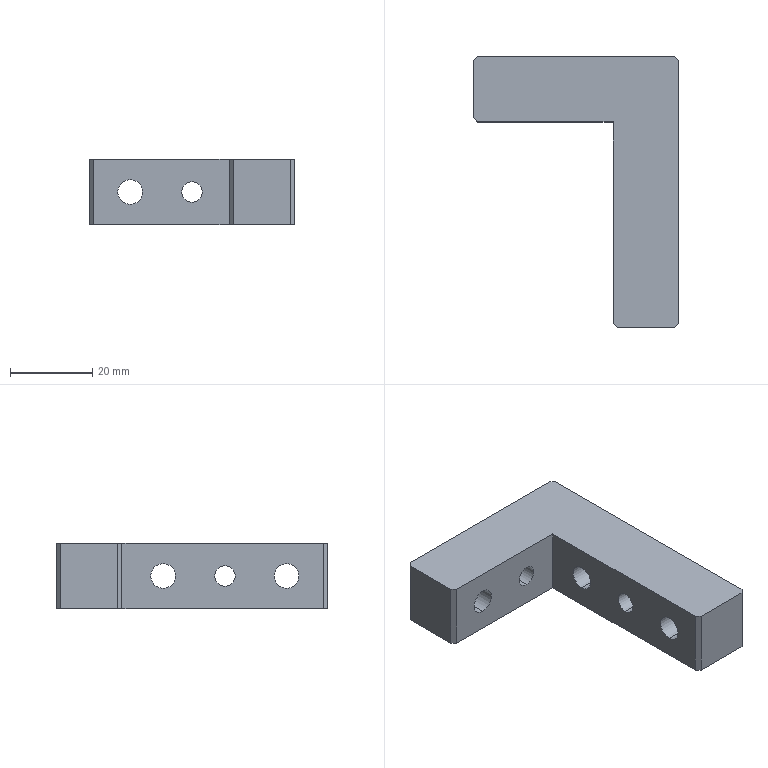Component | SolidWorks | AdjustmentSeat001-1 | 1 solid | 27 faces | box 50 x 66 x 16 mm | volume 22992 mm3 | plane 13 | cylinder 12 | cone 2 | commonest cylinder face diameters 6 x8 5 x4 | material Plain Carbon Steel
build123d program:
from build123d import *

# Parameters (mm, degrees)
EXTRUDE_THIN1_DEPTH          = 8
M6_TAPPED_HOLE2_D            = 5
M6_TAPPED_HOLE2_DEPTH        = 21
M6_TAPPED_HOLE2_TIP          = 1.502
F_6_0_6_DIAMETER_HOLE1_D     = 6
M6_TAPPED_HOLE1_D            = 5
F_6_0_6_DIAMETER_HOLE2_D     = 6
F_6_0_6_DIAMETER_HOLE2_DEPTH = 20
F_6_0_6_DIAMETER_HOLE2_TIP   = 1.803
CHAMFER1_SIZE                = 1


with BuildPart() as part:
    # Sketch1 → Extrude-Thin1 (new, symmetric)
    with BuildSketch(Plane.XY):
        Polygon((0, 34), (0, 0), (-50, 0), (-50, -16), (16, -16), (16, 34), align=None)
    extrude(amount=EXTRUDE_THIN1_DEPTH, both=True)

    # M6 Tapped Hole2
    with Locations(Plane(origin=(0, 0, 0), x_dir=(1, 0, 0), z_dir=(0, 1, 0))):
        with Locations((-25, 0)):
            Hole(M6_TAPPED_HOLE2_D / 2, depth=M6_TAPPED_HOLE2_DEPTH)
            with Locations((0, 0, -(M6_TAPPED_HOLE2_DEPTH + M6_TAPPED_HOLE2_TIP / 2))):  # 118° drill point
                Cone(0, M6_TAPPED_HOLE2_D / 2, M6_TAPPED_HOLE2_TIP, mode=Mode.SUBTRACT)

    # 6.0 _6_ Diameter Hole1 (through all)
    with Locations(Plane(origin=(0, 0, 0), x_dir=(1, 0, 0), z_dir=(0, 1, 0))):
        with Locations((-40, 0), (-10, 0)):
            Hole(F_6_0_6_DIAMETER_HOLE1_D / 2)

    # M6 Tapped Hole1 (through all)
    with Locations(Plane(origin=(16, 0, 0), x_dir=(0, 0, -1), z_dir=(1, 0, 0))):
        with Locations((0, 9)):
            Hole(M6_TAPPED_HOLE1_D / 2)

    # 6.0 _6_ Diameter Hole2
    with Locations(Plane(origin=(16, 0, 0), x_dir=(0, 0, -1), z_dir=(1, 0, 0))):
        with Locations((0, -6), (0, 24)):
            Hole(F_6_0_6_DIAMETER_HOLE2_D / 2, depth=F_6_0_6_DIAMETER_HOLE2_DEPTH)
            with Locations((0, 0, -(F_6_0_6_DIAMETER_HOLE2_DEPTH + F_6_0_6_DIAMETER_HOLE2_TIP / 2))):  # 118° drill point
                Cone(0, F_6_0_6_DIAMETER_HOLE2_D / 2, F_6_0_6_DIAMETER_HOLE2_TIP, mode=Mode.SUBTRACT)

    # Chamfer1
    chamfer1_edges = [part.edges().sort_by_distance(p)[0] for p in [
        (16, -16, 0),
        (-50, -16, 0),
        (-50, 0, 0),
        (0, 34, 0),
        (16, 34, 0),
    ]]
    chamfer(chamfer1_edges, length=CHAMFER1_SIZE)


solid = part.part

# Placed as in the assembly
solid = solid.moved(Location((-17.972, 9.101, 117.932), (0, 0, 90)))
STEP:
#1=COLOUR_RGB('',0.7922,0.8196,0.9333);
#2=FILL_AREA_STYLE_COLOUR('',#1);
#3=FILL_AREA_STYLE('',(#2));
#4=SURFACE_STYLE_FILL_AREA(#3);
#5=SURFACE_SIDE_STYLE('',(#4));
#6=SURFACE_STYLE_USAGE(.BOTH.,#5);
#7=PRESENTATION_STYLE_ASSIGNMENT((#6));
#8=CARTESIAN_POINT('',(-0.4713,0.2008,4.761));
#9=VERTEX_POINT('',#8);
#10=CARTESIAN_POINT('',(-0.4713,0.2008,4.525));
#11=VERTEX_POINT('',#10);
#12=CARTESIAN_POINT('',(-0.4713,0.2008,4.643));
#13=DIRECTION('',(-0.,1.,0.));
#14=DIRECTION('',(0.,0.,-1.));
#15=AXIS2_PLACEMENT_3D('',#12,#13,#14);
#16=CIRCLE('',#15,0.1181);
#17=EDGE_CURVE('',#9,#11,#16,.T.);
#18=ORIENTED_EDGE('',*,*,#17,.F.);
#19=CARTESIAN_POINT('',(-0.4713,0.9882,4.761));
#20=VERTEX_POINT('',#19);
#21=CARTESIAN_POINT('',(-0.4713,0.9882,4.761));
#22=DIRECTION('',(-0.,1.,0.));
#23=VECTOR('',#22,39.37);
#24=LINE('',#21,#23);
#25=EDGE_CURVE('',#9,#20,#24,.T.);
#26=ORIENTED_EDGE('',*,*,#25,.T.);
#27=CARTESIAN_POINT('',(-0.4713,0.9882,4.525));
#28=VERTEX_POINT('',#27);
#29=CARTESIAN_POINT('',(-0.4713,0.9882,4.643));
#30=DIRECTION('',(-0.,1.,0.));
#31=DIRECTION('',(0.,0.,-1.));
#32=AXIS2_PLACEMENT_3D('',#29,#30,#31);
#33=CIRCLE('',#32,0.1181);
#34=EDGE_CURVE('',#20,#28,#33,.T.);
#35=ORIENTED_EDGE('',*,*,#34,.T.);
#36=CARTESIAN_POINT('',(-0.4713,0.9882,4.525));
#37=DIRECTION('',(-0.,1.,0.));
#38=VECTOR('',#37,39.37);
#39=LINE('',#36,#38);
#40=EDGE_CURVE('',#11,#28,#39,.T.);
#41=ORIENTED_EDGE('',*,*,#40,.F.);
#42=EDGE_LOOP('',(#18,#26,#35,#41));
#43=FACE_OUTER_BOUND('',#42,.T.);
#44=CARTESIAN_POINT('',(-0.4713,0.9882,4.643));
#45=DIRECTION('',(-0.,1.,0.));
#46=DIRECTION('',(0.,0.,-1.));
#47=AXIS2_PLACEMENT_3D('',#44,#45,#46);
#48=CYLINDRICAL_SURFACE('',#47,0.1181);
#49=ADVANCED_FACE('',(#43),#48,.F.);
#50=CARTESIAN_POINT('',(-0.4713,0.1299,4.643));
#51=VERTEX_POINT('',#50);
#52=CARTESIAN_POINT('',(-0.4713,0.2008,4.525));
#53=DIRECTION('',(-0.,0.515,-0.8572));
#54=VECTOR('',#53,39.37);
#55=LINE('',#52,#54);
#56=EDGE_CURVE('',#51,#11,#55,.T.);
#57=ORIENTED_EDGE('',*,*,#56,.F.);
#58=CARTESIAN_POINT('',(-0.4713,0.2008,4.761));
#59=DIRECTION('',(-0.,0.515,0.8572));
#60=VECTOR('',#59,39.37);
#61=LINE('',#58,#60);
#62=EDGE_CURVE('',#51,#9,#61,.T.);
#63=ORIENTED_EDGE('',*,*,#62,.T.);
#64=ORIENTED_EDGE('',*,*,#17,.T.);
#65=EDGE_LOOP('',(#57,#63,#64));
#66=FACE_OUTER_BOUND('',#65,.T.);
#67=CARTESIAN_POINT('',(-0.4713,0.2008,4.643));
#68=DIRECTION('',(-0.,1.,0.));
#69=DIRECTION('',(0.,0.,-1.));
#70=AXIS2_PLACEMENT_3D('',#67,#68,#69);
#71=CONICAL_SURFACE('',#70,0.1181,1.03);
#72=ADVANCED_FACE('',(#66),#71,.F.);
#73=CARTESIAN_POINT('',(-1.652,0.3583,4.525));
#74=VERTEX_POINT('',#73);
#75=CARTESIAN_POINT('',(-1.652,0.3583,4.761));
#76=VERTEX_POINT('',#75);
#77=CARTESIAN_POINT('',(-1.652,0.3583,4.643));
#78=DIRECTION('',(0.,-1.,0.));
#79=DIRECTION('',(0.,0.,1.));
#80=AXIS2_PLACEMENT_3D('',#77,#78,#79);
#81=CIRCLE('',#80,0.1181);
#82=EDGE_CURVE('',#74,#76,#81,.T.);
#83=ORIENTED_EDGE('',*,*,#82,.T.);
#84=CARTESIAN_POINT('',(-1.652,0.9882,4.761));
#85=VERTEX_POINT('',#84);
#86=CARTESIAN_POINT('',(-1.652,0.9882,4.761));
#87=DIRECTION('',(-0.,1.,0.));
#88=VECTOR('',#87,39.37);
#89=LINE('',#86,#88);
#90=EDGE_CURVE('',#76,#85,#89,.T.);
#91=ORIENTED_EDGE('',*,*,#90,.T.);
#92=CARTESIAN_POINT('',(-1.652,0.9882,4.525));
#93=VERTEX_POINT('',#92);
#94=CARTESIAN_POINT('',(-1.652,0.9882,4.643));
#95=DIRECTION('',(-0.,1.,0.));
#96=DIRECTION('',(0.,0.,-1.));
#97=AXIS2_PLACEMENT_3D('',#94,#95,#96);
#98=CIRCLE('',#97,0.1181);
#99=EDGE_CURVE('',#85,#93,#98,.T.);
#100=ORIENTED_EDGE('',*,*,#99,.T.);
#101=CARTESIAN_POINT('',(-1.652,0.9882,4.525));
#102=DIRECTION('',(-0.,1.,0.));
#103=VECTOR('',#102,39.37);
#104=LINE('',#101,#103);
#105=EDGE_CURVE('',#74,#93,#104,.T.);
#106=ORIENTED_EDGE('',*,*,#105,.F.);
#107=EDGE_LOOP('',(#83,#91,#100,#106));
#108=FACE_OUTER_BOUND('',#107,.T.);
#109=CARTESIAN_POINT('',(-1.652,0.9882,4.643));
#110=DIRECTION('',(-0.,1.,0.));
#111=DIRECTION('',(0.,0.,-1.));
#112=AXIS2_PLACEMENT_3D('',#109,#110,#111);
#113=CYLINDRICAL_SURFACE('',#112,0.1181);
#114=ADVANCED_FACE('',(#108),#113,.F.);
#115=CARTESIAN_POINT('',(-1.062,0.3583,4.545));
#116=VERTEX_POINT('',#115);
#117=CARTESIAN_POINT('',(-1.062,0.3583,4.741));
#118=VERTEX_POINT('',#117);
#119=CARTESIAN_POINT('',(-1.062,0.3583,4.643));
#120=DIRECTION('',(0.,-1.,0.));
#121=DIRECTION('',(0.,0.,1.));
#122=AXIS2_PLACEMENT_3D('',#119,#120,#121);
#123=CIRCLE('',#122,0.09843);
#124=EDGE_CURVE('',#116,#118,#123,.T.);
#125=ORIENTED_EDGE('',*,*,#124,.T.);
#126=CARTESIAN_POINT('',(-1.062,0.9882,4.741));
#127=VERTEX_POINT('',#126);
#128=CARTESIAN_POINT('',(-1.062,0.9882,4.741));
#129=DIRECTION('',(-0.,1.,0.));
#130=VECTOR('',#129,39.37);
#131=LINE('',#128,#130);
#132=EDGE_CURVE('',#118,#127,#131,.T.);
#133=ORIENTED_EDGE('',*,*,#132,.T.);
#134=CARTESIAN_POINT('',(-1.062,0.9882,4.545));
#135=VERTEX_POINT('',#134);
#136=CARTESIAN_POINT('',(-1.062,0.9882,4.643));
#137=DIRECTION('',(-0.,1.,0.));
#138=DIRECTION('',(0.,0.,-1.));
#139=AXIS2_PLACEMENT_3D('',#136,#137,#138);
#140=CIRCLE('',#139,0.09843);
#141=EDGE_CURVE('',#127,#135,#140,.T.);
#142=ORIENTED_EDGE('',*,*,#141,.T.);
#143=CARTESIAN_POINT('',(-1.062,0.9882,4.545));
#144=DIRECTION('',(-0.,1.,0.));
#145=VECTOR('',#144,39.37);
#146=LINE('',#143,#145);
#147=EDGE_CURVE('',#116,#135,#146,.T.);
#148=ORIENTED_EDGE('',*,*,#147,.F.);
#149=EDGE_LOOP('',(#125,#133,#142,#148));
#150=FACE_OUTER_BOUND('',#149,.T.);
#151=CARTESIAN_POINT('',(-1.062,0.9882,4.643));
#152=DIRECTION('',(-0.,1.,0.));
#153=DIRECTION('',(0.,0.,-1.));
#154=AXIS2_PLACEMENT_3D('',#151,#152,#153);
#155=CYLINDRICAL_SURFACE('',#154,0.09843);
#156=ADVANCED_FACE('',(#150),#155,.F.);
#157=CARTESIAN_POINT('',(-0.07764,-1.216,4.525));
#158=VERTEX_POINT('',#157);
#159=CARTESIAN_POINT('',(-0.07764,-1.216,4.761));
#160=VERTEX_POINT('',#159);
#161=CARTESIAN_POINT('',(-0.07764,-1.216,4.643));
#162=DIRECTION('',(-1.,-0.,0.));
#163=DIRECTION('',(0.,0.,1.));
#164=AXIS2_PLACEMENT_3D('',#161,#162,#163);
#165=CIRCLE('',#164,0.1181);
#166=EDGE_CURVE('',#158,#160,#165,.T.);
#167=ORIENTED_EDGE('',*,*,#166,.F.);
#168=CARTESIAN_POINT('',(-0.7076,-1.216,4.525));
#169=VERTEX_POINT('',#168);
#170=CARTESIAN_POINT('',(-0.7076,-1.216,4.525));
#171=DIRECTION('',(-1.,-0.,0.));
#172=VECTOR('',#171,39.37);
#173=LINE('',#170,#172);
#174=EDGE_CURVE('',#158,#169,#173,.T.);
#175=ORIENTED_EDGE('',*,*,#174,.T.);
#176=CARTESIAN_POINT('',(-0.7076,-1.216,4.761));
#177=VERTEX_POINT('',#176);
#178=CARTESIAN_POINT('',(-0.7076,-1.216,4.643));
#179=DIRECTION('',(-1.,-0.,0.));
#180=DIRECTION('',(0.,0.,1.));
#181=AXIS2_PLACEMENT_3D('',#178,#179,#180);
#182=CIRCLE('',#181,0.1181);
#183=EDGE_CURVE('',#169,#177,#182,.T.);
#184=ORIENTED_EDGE('',*,*,#183,.T.);
#185=CARTESIAN_POINT('',(-0.7076,-1.216,4.761));
#186=DIRECTION('',(-1.,-0.,0.));
#187=VECTOR('',#186,39.37);
#188=LINE('',#185,#187);
#189=EDGE_CURVE('',#160,#177,#188,.T.);
#190=ORIENTED_EDGE('',*,*,#189,.F.);
#191=EDGE_LOOP('',(#167,#175,#184,#190));
#192=FACE_OUTER_BOUND('',#191,.T.);
#193=CARTESIAN_POINT('',(-0.7076,-1.216,4.643));
#194=DIRECTION('',(-1.,-0.,0.));
#195=DIRECTION('',(0.,0.,1.));
#196=AXIS2_PLACEMENT_3D('',#193,#194,#195);
#197=CYLINDRICAL_SURFACE('',#196,0.1181);
#198=ADVANCED_FACE('',(#192),#197,.F.);
#199=CARTESIAN_POINT('',(-0.07764,-0.03539,4.525));
#200=VERTEX_POINT('',#199);
#201=CARTESIAN_POINT('',(-0.07764,-0.03539,4.761));
#202=VERTEX_POINT('',#201);
#203=CARTESIAN_POINT('',(-0.07764,-0.03539,4.643));
#204=DIRECTION('',(-1.,-0.,0.));
#205=DIRECTION('',(0.,0.,1.));
#206=AXIS2_PLACEMENT_3D('',#203,#204,#205);
#207=CIRCLE('',#206,0.1181);
#208=EDGE_CURVE('',#200,#202,#207,.T.);
#209=ORIENTED_EDGE('',*,*,#208,.F.);
#210=CARTESIAN_POINT('',(-0.7076,-0.03539,4.525));
#211=VERTEX_POINT('',#210);
#212=CARTESIAN_POINT('',(-0.7076,-0.03539,4.525));
#213=DIRECTION('',(-1.,-0.,0.));
#214=VECTOR('',#213,39.37);
#215=LINE('',#212,#214);
#216=EDGE_CURVE('',#200,#211,#215,.T.);
#217=ORIENTED_EDGE('',*,*,#216,.T.);
#218=CARTESIAN_POINT('',(-0.7076,-0.03539,4.761));
#219=VERTEX_POINT('',#218);
#220=CARTESIAN_POINT('',(-0.7076,-0.03539,4.643));
#221=DIRECTION('',(-1.,-0.,0.));
#222=DIRECTION('',(0.,0.,1.));
#223=AXIS2_PLACEMENT_3D('',#220,#221,#222);
#224=CIRCLE('',#223,0.1181);
#225=EDGE_CURVE('',#211,#219,#224,.T.);
#226=ORIENTED_EDGE('',*,*,#225,.T.);
#227=CARTESIAN_POINT('',(-0.7076,-0.03539,4.761));
#228=DIRECTION('',(-1.,-0.,0.));
#229=VECTOR('',#228,39.37);
#230=LINE('',#227,#229);
#231=EDGE_CURVE('',#202,#219,#230,.T.);
#232=ORIENTED_EDGE('',*,*,#231,.F.);
#233=EDGE_LOOP('',(#209,#217,#226,#232));
#234=FACE_OUTER_BOUND('',#233,.T.);
#235=CARTESIAN_POINT('',(-0.7076,-0.03539,4.643));
#236=DIRECTION('',(-1.,-0.,0.));
#237=DIRECTION('',(0.,0.,1.));
#238=AXIS2_PLACEMENT_3D('',#235,#236,#237);
#239=CYLINDRICAL_SURFACE('',#238,0.1181);
#240=ADVANCED_FACE('',(#234),#239,.F.);
#241=CARTESIAN_POINT('',(-0.07764,-0.6259,4.545));
#242=VERTEX_POINT('',#241);
#243=CARTESIAN_POINT('',(-0.07764,-0.6259,4.741));
#244=VERTEX_POINT('',#243);
#245=CARTESIAN_POINT('',(-0.07764,-0.6259,4.643));
#246=DIRECTION('',(-1.,-0.,0.));
#247=DIRECTION('',(0.,0.,1.));
#248=AXIS2_PLACEMENT_3D('',#245,#246,#247);
#249=CIRCLE('',#248,0.09843);
#250=EDGE_CURVE('',#242,#244,#249,.T.);
#251=ORIENTED_EDGE('',*,*,#250,.F.);
#252=CARTESIAN_POINT('',(-0.7076,-0.6259,4.545));
#253=VERTEX_POINT('',#252);
#254=CARTESIAN_POINT('',(-0.7076,-0.6259,4.545));
#255=DIRECTION('',(-1.,-0.,0.));
#256=VECTOR('',#255,39.37);
#257=LINE('',#254,#256);
#258=EDGE_CURVE('',#242,#253,#257,.T.);
#259=ORIENTED_EDGE('',*,*,#258,.T.);
#260=CARTESIAN_POINT('',(-0.7076,-0.6259,4.741));
#261=VERTEX_POINT('',#260);
#262=CARTESIAN_POINT('',(-0.7076,-0.6259,4.643));
#263=DIRECTION('',(-1.,-0.,0.));
#264=DIRECTION('',(0.,0.,1.));
#265=AXIS2_PLACEMENT_3D('',#262,#263,#264);
#266=CIRCLE('',#265,0.09843);
#267=EDGE_CURVE('',#253,#261,#266,.T.);
#268=ORIENTED_EDGE('',*,*,#267,.T.);
#269=CARTESIAN_POINT('',(-0.7076,-0.6259,4.741));
#270=DIRECTION('',(-1.,-0.,0.));
#271=VECTOR('',#270,39.37);
#272=LINE('',#269,#271);
#273=EDGE_CURVE('',#244,#261,#272,.T.);
#274=ORIENTED_EDGE('',*,*,#273,.F.);
#275=EDGE_LOOP('',(#251,#259,#268,#274));
#276=FACE_OUTER_BOUND('',#275,.T.);
#277=CARTESIAN_POINT('',(-0.7076,-0.6259,4.643));
#278=DIRECTION('',(-1.,-0.,0.));
#279=DIRECTION('',(0.,0.,1.));
#280=AXIS2_PLACEMENT_3D('',#277,#278,#279);
#281=CYLINDRICAL_SURFACE('',#280,0.09843);
#282=ADVANCED_FACE('',(#276),#281,.F.);
#283=CARTESIAN_POINT('',(-0.4713,0.9882,4.643));
#284=DIRECTION('',(-0.,1.,0.));
#285=DIRECTION('',(0.,0.,-1.));
#286=AXIS2_PLACEMENT_3D('',#283,#284,#285);
#287=CIRCLE('',#286,0.1181);
#288=EDGE_CURVE('',#28,#20,#287,.T.);
#289=ORIENTED_EDGE('',*,*,#288,.F.);
#290=ORIENTED_EDGE('',*,*,#34,.F.);
#291=EDGE_LOOP('',(#289,#290));
#292=FACE_BOUND('',#291,.T.);
#293=CARTESIAN_POINT('',(-1.652,0.9882,4.643));
#294=DIRECTION('',(-0.,1.,0.));
#295=DIRECTION('',(0.,0.,-1.));
#296=AXIS2_PLACEMENT_3D('',#293,#294,#295);
#297=CIRCLE('',#296,0.1181);
#298=EDGE_CURVE('',#93,#85,#297,.T.);
#299=ORIENTED_EDGE('',*,*,#298,.F.);
#300=ORIENTED_EDGE('',*,*,#99,.F.);
#301=EDGE_LOOP('',(#299,#300));
#302=FACE_BOUND('',#301,.T.);
#303=CARTESIAN_POINT('',(-1.062,0.9882,4.643));
#304=DIRECTION('',(-0.,1.,0.));
#305=DIRECTION('',(0.,0.,-1.));
#306=AXIS2_PLACEMENT_3D('',#303,#304,#305);
#307=CIRCLE('',#306,0.09843);
#308=EDGE_CURVE('',#135,#127,#307,.T.);
#309=ORIENTED_EDGE('',*,*,#308,.F.);
#310=ORIENTED_EDGE('',*,*,#141,.F.);
#311=EDGE_LOOP('',(#309,#310));
#312=FACE_BOUND('',#311,.T.);
#313=CARTESIAN_POINT('',(-0.117,0.9882,4.958));
#314=VERTEX_POINT('',#313);
#315=CARTESIAN_POINT('',(-2.007,0.9882,4.958));
#316=VERTEX_POINT('',#315);
#317=CARTESIAN_POINT('',(-0.7076,0.9882,4.958));
#318=DIRECTION('',(-1.,-0.,0.));
#319=VECTOR('',#318,39.37);
#320=LINE('',#317,#319);
#321=EDGE_CURVE('',#314,#316,#320,.T.);
#322=ORIENTED_EDGE('',*,*,#321,.F.);
#323=CARTESIAN_POINT('',(-0.117,0.9882,4.328));
#324=VERTEX_POINT('',#323);
#325=CARTESIAN_POINT('',(-0.117,0.9882,4.958));
#326=DIRECTION('',(0.,0.,-1.));
#327=VECTOR('',#326,39.37);
#328=LINE('',#325,#327);
#329=EDGE_CURVE('',#314,#324,#328,.T.);
#330=ORIENTED_EDGE('',*,*,#329,.T.);
#331=CARTESIAN_POINT('',(-2.007,0.9882,4.328));
#332=VERTEX_POINT('',#331);
#333=CARTESIAN_POINT('',(-0.7076,0.9882,4.328));
#334=DIRECTION('',(-1.,-0.,0.));
#335=VECTOR('',#334,39.37);
#336=LINE('',#333,#335);
#337=EDGE_CURVE('',#324,#332,#336,.T.);
#338=ORIENTED_EDGE('',*,*,#337,.T.);
#339=CARTESIAN_POINT('',(-2.007,0.9882,4.958));
#340=DIRECTION('',(0.,0.,1.));
#341=VECTOR('',#340,39.37);
#342=LINE('',#339,#341);
#343=EDGE_CURVE('',#332,#316,#342,.T.);
#344=ORIENTED_EDGE('',*,*,#343,.T.);
#345=EDGE_LOOP('',(#322,#330,#338,#344));
#346=FACE_OUTER_BOUND('',#345,.T.);
#347=CARTESIAN_POINT('',(-0.7076,0.9882,4.958));
#348=DIRECTION('',(0.,-1.,0.));
#349=DIRECTION('',(0.,0.,1.));
#350=AXIS2_PLACEMENT_3D('',#347,#348,#349);
#351=PLANE('',#350);
#352=ADVANCED_FACE('',(#292,#302,#312,#346),#351,.F.);
#353=CARTESIAN_POINT('',(-2.046,0.3977,4.958));
#354=VERTEX_POINT('',#353);
#355=CARTESIAN_POINT('',(-2.046,0.9489,4.958));
#356=VERTEX_POINT('',#355);
#357=CARTESIAN_POINT('',(-2.046,0.3583,4.958));
#358=DIRECTION('',(-0.,1.,0.));
#359=VECTOR('',#358,39.37);
#360=LINE('',#357,#359);
#361=EDGE_CURVE('',#354,#356,#360,.T.);
#362=ORIENTED_EDGE('',*,*,#361,.T.);
#363=CARTESIAN_POINT('',(-2.046,0.9489,4.328));
#364=VERTEX_POINT('',#363);
#365=CARTESIAN_POINT('',(-2.046,0.9489,4.328));
#366=DIRECTION('',(0.,0.,-1.));
#367=VECTOR('',#366,39.37);
#368=LINE('',#365,#367);
#369=EDGE_CURVE('',#356,#364,#368,.T.);
#370=ORIENTED_EDGE('',*,*,#369,.T.);
#371=CARTESIAN_POINT('',(-2.046,0.3977,4.328));
#372=VERTEX_POINT('',#371);
#373=CARTESIAN_POINT('',(-2.046,0.3583,4.328));
#374=DIRECTION('',(-0.,1.,0.));
#375=VECTOR('',#374,39.37);
#376=LINE('',#373,#375);
#377=EDGE_CURVE('',#372,#364,#376,.T.);
#378=ORIENTED_EDGE('',*,*,#377,.F.);
#379=CARTESIAN_POINT('',(-2.046,0.3977,4.958));
#380=DIRECTION('',(0.,0.,1.));
#381=VECTOR('',#380,39.37);
#382=LINE('',#379,#381);
#383=EDGE_CURVE('',#372,#354,#382,.T.);
#384=ORIENTED_EDGE('',*,*,#383,.T.);
#385=EDGE_LOOP('',(#362,#370,#378,#384));
#386=FACE_OUTER_BOUND('',#385,.T.);
#387=CARTESIAN_POINT('',(-2.046,0.3583,4.958));
#388=DIRECTION('',(-1.,-0.,0.));
#389=DIRECTION('',(0.,0.,1.));
#390=AXIS2_PLACEMENT_3D('',#387,#388,#389);
#391=PLANE('',#390);
#392=ADVANCED_FACE('',(#386),#391,.T.);
#393=ORIENTED_EDGE('',*,*,#82,.F.);
#394=CARTESIAN_POINT('',(-1.652,0.3583,4.643));
#395=DIRECTION('',(0.,-1.,0.));
#396=DIRECTION('',(0.,0.,1.));
#397=AXIS2_PLACEMENT_3D('',#394,#395,#396);
#398=CIRCLE('',#397,0.1181);
#399=EDGE_CURVE('',#76,#74,#398,.T.);
#400=ORIENTED_EDGE('',*,*,#399,.F.);
#401=EDGE_LOOP('',(#393,#400));
#402=FACE_BOUND('',#401,.T.);
#403=ORIENTED_EDGE('',*,*,#124,.F.);
#404=CARTESIAN_POINT('',(-1.062,0.3583,4.643));
#405=DIRECTION('',(0.,-1.,0.));
#406=DIRECTION('',(0.,0.,1.));
#407=AXIS2_PLACEMENT_3D('',#404,#405,#406);
#408=CIRCLE('',#407,0.09843);
#409=EDGE_CURVE('',#118,#116,#408,.T.);
#410=ORIENTED_EDGE('',*,*,#409,.F.);
#411=EDGE_LOOP('',(#403,#410));
#412=FACE_BOUND('',#411,.T.);
#413=CARTESIAN_POINT('',(-0.7076,0.3583,4.958));
#414=VERTEX_POINT('',#413);
#415=CARTESIAN_POINT('',(-2.007,0.3583,4.958));
#416=VERTEX_POINT('',#415);
#417=CARTESIAN_POINT('',(-0.7076,0.3583,4.958));
#418=DIRECTION('',(-1.,-0.,0.));
#419=VECTOR('',#418,39.37);
#420=LINE('',#417,#419);
#421=EDGE_CURVE('',#414,#416,#420,.T.);
#422=ORIENTED_EDGE('',*,*,#421,.T.);
#423=CARTESIAN_POINT('',(-2.007,0.3583,4.328));
#424=VERTEX_POINT('',#423);
#425=CARTESIAN_POINT('',(-2.007,0.3583,4.958));
#426=DIRECTION('',(0.,0.,-1.));
#427=VECTOR('',#426,39.37);
#428=LINE('',#425,#427);
#429=EDGE_CURVE('',#416,#424,#428,.T.);
#430=ORIENTED_EDGE('',*,*,#429,.T.);
#431=CARTESIAN_POINT('',(-0.7076,0.3583,4.328));
#432=VERTEX_POINT('',#431);
#433=CARTESIAN_POINT('',(-0.7076,0.3583,4.328));
#434=DIRECTION('',(-1.,-0.,0.));
#435=VECTOR('',#434,39.37);
#436=LINE('',#433,#435);
#437=EDGE_CURVE('',#432,#424,#436,.T.);
#438=ORIENTED_EDGE('',*,*,#437,.F.);
#439=CARTESIAN_POINT('',(-0.7076,0.3583,4.958));
#440=DIRECTION('',(0.,0.,-1.));
#441=VECTOR('',#440,39.37);
#442=LINE('',#439,#441);
#443=EDGE_CURVE('',#414,#432,#442,.T.);
#444=ORIENTED_EDGE('',*,*,#443,.F.);
#445=EDGE_LOOP('',(#422,#430,#438,#444));
#446=FACE_OUTER_BOUND('',#445,.T.);
#447=CARTESIAN_POINT('',(-0.7076,0.3583,4.958));
#448=DIRECTION('',(0.,-1.,0.));
#449=DIRECTION('',(0.,0.,1.));
#450=AXIS2_PLACEMENT_3D('',#447,#448,#449);
#451=PLANE('',#450);
#452=ADVANCED_FACE('',(#402,#412,#446),#451,.T.);
#453=CARTESIAN_POINT('',(-0.7076,-1.216,4.643));
#454=DIRECTION('',(-1.,-0.,0.));
#455=DIRECTION('',(0.,0.,1.));
#456=AXIS2_PLACEMENT_3D('',#453,#454,#455);
#457=CIRCLE('',#456,0.1181);
#458=EDGE_CURVE('',#177,#169,#457,.T.);
#459=ORIENTED_EDGE('',*,*,#458,.F.);
#460=ORIENTED_EDGE('',*,*,#183,.F.);
#461=EDGE_LOOP('',(#459,#460));
#462=FACE_BOUND('',#461,.T.);
#463=CARTESIAN_POINT('',(-0.7076,-0.03539,4.643));
#464=DIRECTION('',(-1.,-0.,0.));
#465=DIRECTION('',(0.,0.,1.));
#466=AXIS2_PLACEMENT_3D('',#463,#464,#465);
#467=CIRCLE('',#466,0.1181);
#468=EDGE_CURVE('',#219,#211,#467,.T.);
#469=ORIENTED_EDGE('',*,*,#468,.F.);
#470=ORIENTED_EDGE('',*,*,#225,.F.);
#471=EDGE_LOOP('',(#469,#470));
#472=FACE_BOUND('',#471,.T.);
#473=CARTESIAN_POINT('',(-0.7076,-0.6259,4.643));
#474=DIRECTION('',(-1.,-0.,0.));
#475=DIRECTION('',(0.,0.,1.));
#476=AXIS2_PLACEMENT_3D('',#473,#474,#475);
#477=CIRCLE('',#476,0.09843);
#478=EDGE_CURVE('',#261,#253,#477,.T.);
#479=ORIENTED_EDGE('',*,*,#478,.F.);
#480=ORIENTED_EDGE('',*,*,#267,.F.);
#481=EDGE_LOOP('',(#479,#480));
#482=FACE_BOUND('',#481,.T.);
#483=CARTESIAN_POINT('',(-0.7076,-1.571,4.328));
#484=VERTEX_POINT('',#483);
#485=CARTESIAN_POINT('',(-0.7076,0.3583,4.328));
#486=DIRECTION('',(-0.,1.,0.));
#487=VECTOR('',#486,39.37);
#488=LINE('',#485,#487);
#489=EDGE_CURVE('',#484,#432,#488,.T.);
#490=ORIENTED_EDGE('',*,*,#489,.F.);
#491=CARTESIAN_POINT('',(-0.7076,-1.571,4.958));
#492=VERTEX_POINT('',#491);
#493=CARTESIAN_POINT('',(-0.7076,-1.571,4.958));
#494=DIRECTION('',(0.,0.,1.));
#495=VECTOR('',#494,39.37);
#496=LINE('',#493,#495);
#497=EDGE_CURVE('',#484,#492,#496,.T.);
#498=ORIENTED_EDGE('',*,*,#497,.T.);
#499=CARTESIAN_POINT('',(-0.7076,0.3583,4.958));
#500=DIRECTION('',(-0.,1.,0.));
#501=VECTOR('',#500,39.37);
#502=LINE('',#499,#501);
#503=EDGE_CURVE('',#492,#414,#502,.T.);
#504=ORIENTED_EDGE('',*,*,#503,.T.);
#505=ORIENTED_EDGE('',*,*,#443,.T.);
#506=EDGE_LOOP('',(#490,#498,#504,#505));
#507=FACE_OUTER_BOUND('',#506,.T.);
#508=CARTESIAN_POINT('',(-0.7076,0.3583,4.958));
#509=DIRECTION('',(-1.,-0.,0.));
#510=DIRECTION('',(0.,0.,1.));
#511=AXIS2_PLACEMENT_3D('',#508,#509,#510);
#512=PLANE('',#511);
#513=ADVANCED_FACE('',(#462,#472,#482,#507),#512,.T.);
#514=CARTESIAN_POINT('',(-0.117,-1.61,4.328));
#515=VERTEX_POINT('',#514);
#516=CARTESIAN_POINT('',(-0.6682,-1.61,4.328));
#517=VERTEX_POINT('',#516);
#518=CARTESIAN_POINT('',(-0.07764,-1.61,4.328));
#519=DIRECTION('',(-1.,-0.,0.));
#520=VECTOR('',#519,39.37);
#521=LINE('',#518,#520);
#522=EDGE_CURVE('',#515,#517,#521,.T.);
#523=ORIENTED_EDGE('',*,*,#522,.F.);
#524=CARTESIAN_POINT('',(-0.117,-1.61,4.958));
#525=VERTEX_POINT('',#524);
#526=CARTESIAN_POINT('',(-0.117,-1.61,4.958));
#527=DIRECTION('',(0.,0.,1.));
#528=VECTOR('',#527,39.37);
#529=LINE('',#526,#528);
#530=EDGE_CURVE('',#515,#525,#529,.T.);
#531=ORIENTED_EDGE('',*,*,#530,.T.);
#532=CARTESIAN_POINT('',(-0.6682,-1.61,4.958));
#533=VERTEX_POINT('',#532);
#534=CARTESIAN_POINT('',(-0.07764,-1.61,4.958));
#535=DIRECTION('',(-1.,-0.,0.));
#536=VECTOR('',#535,39.37);
#537=LINE('',#534,#536);
#538=EDGE_CURVE('',#525,#533,#537,.T.);
#539=ORIENTED_EDGE('',*,*,#538,.T.);
#540=CARTESIAN_POINT('',(-0.6682,-1.61,4.958));
#541=DIRECTION('',(0.,0.,-1.));
#542=VECTOR('',#541,39.37);
#543=LINE('',#540,#542);
#544=EDGE_CURVE('',#533,#517,#543,.T.);
#545=ORIENTED_EDGE('',*,*,#544,.T.);
#546=EDGE_LOOP('',(#523,#531,#539,#545));
#547=FACE_OUTER_BOUND('',#546,.T.);
#548=CARTESIAN_POINT('',(-0.07764,-1.61,4.958));
#549=DIRECTION('',(0.,-1.,0.));
#550=DIRECTION('',(0.,0.,1.));
#551=AXIS2_PLACEMENT_3D('',#548,#549,#550);
#552=PLANE('',#551);
#553=ADVANCED_FACE('',(#547),#552,.T.);
#554=CARTESIAN_POINT('',(-0.07764,-1.216,4.643));
#555=DIRECTION('',(-1.,-0.,0.));
#556=DIRECTION('',(0.,0.,1.));
#557=AXIS2_PLACEMENT_3D('',#554,#555,#556);
#558=CIRCLE('',#557,0.1181);
#559=EDGE_CURVE('',#160,#158,#558,.T.);
#560=ORIENTED_EDGE('',*,*,#559,.T.);
#561=ORIENTED_EDGE('',*,*,#166,.T.);
#562=EDGE_LOOP('',(#560,#561));
#563=FACE_BOUND('',#562,.T.);
#564=CARTESIAN_POINT('',(-0.07764,-0.03539,4.643));
#565=DIRECTION('',(-1.,-0.,0.));
#566=DIRECTION('',(0.,0.,1.));
#567=AXIS2_PLACEMENT_3D('',#564,#565,#566);
#568=CIRCLE('',#567,0.1181);
#569=EDGE_CURVE('',#202,#200,#568,.T.);
#570=ORIENTED_EDGE('',*,*,#569,.T.);
#571=ORIENTED_EDGE('',*,*,#208,.T.);
#572=EDGE_LOOP('',(#570,#571));
#573=FACE_BOUND('',#572,.T.);
#574=CARTESIAN_POINT('',(-0.07764,-0.6259,4.643));
#575=DIRECTION('',(-1.,-0.,0.));
#576=DIRECTION('',(0.,0.,1.));
#577=AXIS2_PLACEMENT_3D('',#574,#575,#576);
#578=CIRCLE('',#577,0.09843);
#579=EDGE_CURVE('',#244,#242,#578,.T.);
#580=ORIENTED_EDGE('',*,*,#579,.T.);
#581=ORIENTED_EDGE('',*,*,#250,.T.);
#582=EDGE_LOOP('',(#580,#581));
#583=FACE_BOUND('',#582,.T.);
#584=CARTESIAN_POINT('',(-0.07764,-1.571,4.328));
#585=VERTEX_POINT('',#584);
#586=CARTESIAN_POINT('',(-0.07764,0.9489,4.328));
#587=VERTEX_POINT('',#586);
#588=CARTESIAN_POINT('',(-0.07764,0.3583,4.328));
#589=DIRECTION('',(-0.,1.,0.));
#590=VECTOR('',#589,39.37);
#591=LINE('',#588,#590);
#592=EDGE_CURVE('',#585,#587,#591,.T.);
#593=ORIENTED_EDGE('',*,*,#592,.T.);
#594=CARTESIAN_POINT('',(-0.07764,0.9489,4.958));
#595=VERTEX_POINT('',#594);
#596=CARTESIAN_POINT('',(-0.07764,0.9489,4.958));
#597=DIRECTION('',(0.,0.,1.));
#598=VECTOR('',#597,39.37);
#599=LINE('',#596,#598);
#600=EDGE_CURVE('',#587,#595,#599,.T.);
#601=ORIENTED_EDGE('',*,*,#600,.T.);
#602=CARTESIAN_POINT('',(-0.07764,-1.571,4.958));
#603=VERTEX_POINT('',#602);
#604=CARTESIAN_POINT('',(-0.07764,0.3583,4.958));
#605=DIRECTION('',(-0.,1.,0.));
#606=VECTOR('',#605,39.37);
#607=LINE('',#604,#606);
#608=EDGE_CURVE('',#603,#595,#607,.T.);
#609=ORIENTED_EDGE('',*,*,#608,.F.);
#610=CARTESIAN_POINT('',(-0.07764,-1.571,4.328));
#611=DIRECTION('',(0.,0.,-1.));
#612=VECTOR('',#611,39.37);
#613=LINE('',#610,#612);
#614=EDGE_CURVE('',#603,#585,#613,.T.);
#615=ORIENTED_EDGE('',*,*,#614,.T.);
#616=EDGE_LOOP('',(#593,#601,#609,#615));
#617=FACE_OUTER_BOUND('',#616,.T.);
#618=CARTESIAN_POINT('',(-0.07764,0.3583,4.958));
#619=DIRECTION('',(-1.,-0.,0.));
#620=DIRECTION('',(0.,0.,1.));
#621=AXIS2_PLACEMENT_3D('',#618,#619,#620);
#622=PLANE('',#621);
#623=ADVANCED_FACE('',(#563,#573,#583,#617),#622,.F.);
#624=ORIENTED_EDGE('',*,*,#608,.T.);
#625=CARTESIAN_POINT('',(-0.117,0.9882,4.958));
#626=DIRECTION('',(-0.7071,0.7071,0.));
#627=VECTOR('',#626,39.37);
#628=LINE('',#625,#627);
#629=EDGE_CURVE('',#595,#314,#628,.T.);
#630=ORIENTED_EDGE('',*,*,#629,.T.);
#631=ORIENTED_EDGE('',*,*,#321,.T.);
#632=CARTESIAN_POINT('',(-2.046,0.9489,4.958));
#633=DIRECTION('',(-0.7071,-0.7071,0.));
#634=VECTOR('',#633,39.37);
#635=LINE('',#632,#634);
#636=EDGE_CURVE('',#316,#356,#635,.T.);
#637=ORIENTED_EDGE('',*,*,#636,.T.);
#638=ORIENTED_EDGE('',*,*,#361,.F.);
#639=CARTESIAN_POINT('',(-2.007,0.3583,4.958));
#640=DIRECTION('',(0.7071,-0.7071,0.));
#641=VECTOR('',#640,39.37);
#642=LINE('',#639,#641);
#643=EDGE_CURVE('',#354,#416,#642,.T.);
#644=ORIENTED_EDGE('',*,*,#643,.T.);
#645=ORIENTED_EDGE('',*,*,#421,.F.);
#646=ORIENTED_EDGE('',*,*,#503,.F.);
#647=CARTESIAN_POINT('',(-0.6682,-1.61,4.958));
#648=DIRECTION('',(0.7071,-0.7071,0.));
#649=VECTOR('',#648,39.37);
#650=LINE('',#647,#649);
#651=EDGE_CURVE('',#492,#533,#650,.T.);
#652=ORIENTED_EDGE('',*,*,#651,.T.);
#653=ORIENTED_EDGE('',*,*,#538,.F.);
#654=CARTESIAN_POINT('',(-0.07764,-1.571,4.958));
#655=DIRECTION('',(0.7071,0.7071,0.));
#656=VECTOR('',#655,39.37);
#657=LINE('',#654,#656);
#658=EDGE_CURVE('',#525,#603,#657,.T.);
#659=ORIENTED_EDGE('',*,*,#658,.T.);
#660=EDGE_LOOP('',(#624,#630,#631,#637,#638,#644,#645,#646,#652,#653,#659));
#661=FACE_OUTER_BOUND('',#660,.T.);
#662=CARTESIAN_POINT('',(-0.7076,0.3583,4.958));
#663=DIRECTION('',(0.,0.,-1.));
#664=DIRECTION('',(0.,-1.,0.));
#665=AXIS2_PLACEMENT_3D('',#662,#663,#664);
#666=PLANE('',#665);
#667=ADVANCED_FACE('',(#661),#666,.F.);
#668=ORIENTED_EDGE('',*,*,#337,.F.);
#669=CARTESIAN_POINT('',(-0.09732,0.9685,4.328));
#670=DIRECTION('',(0.7071,-0.7071,0.));
#671=VECTOR('',#670,39.37);
#672=LINE('',#669,#671);
#673=EDGE_CURVE('',#324,#587,#672,.T.);
#674=ORIENTED_EDGE('',*,*,#673,.T.);
#675=ORIENTED_EDGE('',*,*,#592,.F.);
#676=CARTESIAN_POINT('',(0.572,-0.9212,4.328));
#677=DIRECTION('',(-0.7071,-0.7071,0.));
#678=VECTOR('',#677,39.37);
#679=LINE('',#676,#678);
#680=EDGE_CURVE('',#585,#515,#679,.T.);
#681=ORIENTED_EDGE('',*,*,#680,.T.);
#682=ORIENTED_EDGE('',*,*,#522,.T.);
#683=CARTESIAN_POINT('',(-1.672,-0.6063,4.328));
#684=DIRECTION('',(-0.7071,0.7071,0.));
#685=VECTOR('',#684,39.37);
#686=LINE('',#683,#685);
#687=EDGE_CURVE('',#517,#484,#686,.T.);
#688=ORIENTED_EDGE('',*,*,#687,.T.);
#689=ORIENTED_EDGE('',*,*,#489,.T.);
#690=ORIENTED_EDGE('',*,*,#437,.T.);
#691=CARTESIAN_POINT('',(-1.357,-0.2913,4.328));
#692=DIRECTION('',(-0.7071,0.7071,0.));
#693=VECTOR('',#692,39.37);
#694=LINE('',#691,#693);
#695=EDGE_CURVE('',#424,#372,#694,.T.);
#696=ORIENTED_EDGE('',*,*,#695,.T.);
#697=ORIENTED_EDGE('',*,*,#377,.T.);
#698=CARTESIAN_POINT('',(-1.672,1.323,4.328));
#699=DIRECTION('',(0.7071,0.7071,0.));
#700=VECTOR('',#699,39.37);
#701=LINE('',#698,#700);
#702=EDGE_CURVE('',#364,#332,#701,.T.);
#703=ORIENTED_EDGE('',*,*,#702,.T.);
#704=EDGE_LOOP('',(#668,#674,#675,#681,#682,#688,#689,#690,#696,#697,#703));
#705=FACE_OUTER_BOUND('',#704,.T.);
#706=CARTESIAN_POINT('',(-0.7076,0.3583,4.328));
#707=DIRECTION('',(0.,0.,-1.));
#708=DIRECTION('',(0.,-1.,0.));
#709=AXIS2_PLACEMENT_3D('',#706,#707,#708);
#710=PLANE('',#709);
#711=ADVANCED_FACE('',(#705),#710,.T.);
#712=ORIENTED_EDGE('',*,*,#258,.F.);
#713=ORIENTED_EDGE('',*,*,#579,.F.);
#714=ORIENTED_EDGE('',*,*,#273,.T.);
#715=ORIENTED_EDGE('',*,*,#478,.T.);
#716=EDGE_LOOP('',(#712,#713,#714,#715));
#717=FACE_OUTER_BOUND('',#716,.T.);
#718=CARTESIAN_POINT('',(-0.7076,-0.6259,4.643));
#719=DIRECTION('',(-1.,-0.,0.));
#720=DIRECTION('',(0.,0.,1.));
#721=AXIS2_PLACEMENT_3D('',#718,#719,#720);
#722=CYLINDRICAL_SURFACE('',#721,0.09843);
#723=ADVANCED_FACE('',(#717),#722,.F.);
#724=ORIENTED_EDGE('',*,*,#216,.F.);
#725=ORIENTED_EDGE('',*,*,#569,.F.);
#726=ORIENTED_EDGE('',*,*,#231,.T.);
#727=ORIENTED_EDGE('',*,*,#468,.T.);
#728=EDGE_LOOP('',(#724,#725,#726,#727));
#729=FACE_OUTER_BOUND('',#728,.T.);
#730=CARTESIAN_POINT('',(-0.7076,-0.03539,4.643));
#731=DIRECTION('',(-1.,-0.,0.));
#732=DIRECTION('',(0.,0.,1.));
#733=AXIS2_PLACEMENT_3D('',#730,#731,#732);
#734=CYLINDRICAL_SURFACE('',#733,0.1181);
#735=ADVANCED_FACE('',(#729),#734,.F.);
#736=ORIENTED_EDGE('',*,*,#174,.F.);
#737=ORIENTED_EDGE('',*,*,#559,.F.);
#738=ORIENTED_EDGE('',*,*,#189,.T.);
#739=ORIENTED_EDGE('',*,*,#458,.T.);
#740=EDGE_LOOP('',(#736,#737,#738,#739));
#741=FACE_OUTER_BOUND('',#740,.T.);
#742=CARTESIAN_POINT('',(-0.7076,-1.216,4.643));
#743=DIRECTION('',(-1.,-0.,0.));
#744=DIRECTION('',(0.,0.,1.));
#745=AXIS2_PLACEMENT_3D('',#742,#743,#744);
#746=CYLINDRICAL_SURFACE('',#745,0.1181);
#747=ADVANCED_FACE('',(#741),#746,.F.);
#748=ORIENTED_EDGE('',*,*,#132,.F.);
#749=ORIENTED_EDGE('',*,*,#409,.T.);
#750=ORIENTED_EDGE('',*,*,#147,.T.);
#751=ORIENTED_EDGE('',*,*,#308,.T.);
#752=EDGE_LOOP('',(#748,#749,#750,#751));
#753=FACE_OUTER_BOUND('',#752,.T.);
#754=CARTESIAN_POINT('',(-1.062,0.9882,4.643));
#755=DIRECTION('',(-0.,1.,0.));
#756=DIRECTION('',(0.,0.,-1.));
#757=AXIS2_PLACEMENT_3D('',#754,#755,#756);
#758=CYLINDRICAL_SURFACE('',#757,0.09843);
#759=ADVANCED_FACE('',(#753),#758,.F.);
#760=ORIENTED_EDGE('',*,*,#90,.F.);
#761=ORIENTED_EDGE('',*,*,#399,.T.);
#762=ORIENTED_EDGE('',*,*,#105,.T.);
#763=ORIENTED_EDGE('',*,*,#298,.T.);
#764=EDGE_LOOP('',(#760,#761,#762,#763));
#765=FACE_OUTER_BOUND('',#764,.T.);
#766=CARTESIAN_POINT('',(-1.652,0.9882,4.643));
#767=DIRECTION('',(-0.,1.,0.));
#768=DIRECTION('',(0.,0.,-1.));
#769=AXIS2_PLACEMENT_3D('',#766,#767,#768);
#770=CYLINDRICAL_SURFACE('',#769,0.1181);
#771=ADVANCED_FACE('',(#765),#770,.F.);
#772=ORIENTED_EDGE('',*,*,#62,.F.);
#773=ORIENTED_EDGE('',*,*,#56,.T.);
#774=CARTESIAN_POINT('',(-0.4713,0.2008,4.643));
#775=DIRECTION('',(-0.,1.,0.));
#776=DIRECTION('',(0.,0.,-1.));
#777=AXIS2_PLACEMENT_3D('',#774,#775,#776);
#778=CIRCLE('',#777,0.1181);
#779=EDGE_CURVE('',#11,#9,#778,.T.);
#780=ORIENTED_EDGE('',*,*,#779,.T.);
#781=EDGE_LOOP('',(#772,#773,#780));
#782=FACE_OUTER_BOUND('',#781,.T.);
#783=CARTESIAN_POINT('',(-0.4713,0.2008,4.643));
#784=DIRECTION('',(-0.,1.,0.));
#785=DIRECTION('',(0.,0.,-1.));
#786=AXIS2_PLACEMENT_3D('',#783,#784,#785);
#787=CONICAL_SURFACE('',#786,0.1181,1.03);
#788=ADVANCED_FACE('',(#782),#787,.F.);
#789=ORIENTED_EDGE('',*,*,#25,.F.);
#790=ORIENTED_EDGE('',*,*,#779,.F.);
#791=ORIENTED_EDGE('',*,*,#40,.T.);
#792=ORIENTED_EDGE('',*,*,#288,.T.);
#793=EDGE_LOOP('',(#789,#790,#791,#792));
#794=FACE_OUTER_BOUND('',#793,.T.);
#795=CARTESIAN_POINT('',(-0.4713,0.9882,4.643));
#796=DIRECTION('',(-0.,1.,0.));
#797=DIRECTION('',(0.,0.,-1.));
#798=AXIS2_PLACEMENT_3D('',#795,#796,#797);
#799=CYLINDRICAL_SURFACE('',#798,0.1181);
#800=ADVANCED_FACE('',(#794),#799,.F.);
#801=ORIENTED_EDGE('',*,*,#629,.F.);
#802=ORIENTED_EDGE('',*,*,#600,.F.);
#803=ORIENTED_EDGE('',*,*,#673,.F.);
#804=ORIENTED_EDGE('',*,*,#329,.F.);
#805=EDGE_LOOP('',(#801,#802,#803,#804));
#806=FACE_OUTER_BOUND('',#805,.T.);
#807=CARTESIAN_POINT('',(-0.117,0.9882,4.958));
#808=DIRECTION('',(-0.7071,-0.7071,0.));
#809=DIRECTION('',(0.,0.,-1.));
#810=AXIS2_PLACEMENT_3D('',#807,#808,#809);
#811=PLANE('',#810);
#812=ADVANCED_FACE('',(#806),#811,.F.);
#813=ORIENTED_EDGE('',*,*,#636,.F.);
#814=ORIENTED_EDGE('',*,*,#343,.F.);
#815=ORIENTED_EDGE('',*,*,#702,.F.);
#816=ORIENTED_EDGE('',*,*,#369,.F.);
#817=EDGE_LOOP('',(#813,#814,#815,#816));
#818=FACE_OUTER_BOUND('',#817,.T.);
#819=CARTESIAN_POINT('',(-2.046,0.9489,4.958));
#820=DIRECTION('',(-0.7071,0.7071,0.));
#821=DIRECTION('',(0.,0.,1.));
#822=AXIS2_PLACEMENT_3D('',#819,#820,#821);
#823=PLANE('',#822);
#824=ADVANCED_FACE('',(#818),#823,.T.);
#825=ORIENTED_EDGE('',*,*,#643,.F.);
#826=ORIENTED_EDGE('',*,*,#383,.F.);
#827=ORIENTED_EDGE('',*,*,#695,.F.);
#828=ORIENTED_EDGE('',*,*,#429,.F.);
#829=EDGE_LOOP('',(#825,#826,#827,#828));
#830=FACE_OUTER_BOUND('',#829,.T.);
#831=CARTESIAN_POINT('',(-2.007,0.3583,4.958));
#832=DIRECTION('',(0.7071,0.7071,0.));
#833=DIRECTION('',(0.,0.,-1.));
#834=AXIS2_PLACEMENT_3D('',#831,#832,#833);
#835=PLANE('',#834);
#836=ADVANCED_FACE('',(#830),#835,.F.);
#837=ORIENTED_EDGE('',*,*,#658,.F.);
#838=ORIENTED_EDGE('',*,*,#530,.F.);
#839=ORIENTED_EDGE('',*,*,#680,.F.);
#840=ORIENTED_EDGE('',*,*,#614,.F.);
#841=EDGE_LOOP('',(#837,#838,#839,#840));
#842=FACE_OUTER_BOUND('',#841,.T.);
#843=CARTESIAN_POINT('',(-0.07764,-1.571,4.958));
#844=DIRECTION('',(0.7071,-0.7071,0.));
#845=DIRECTION('',(0.,0.,1.));
#846=AXIS2_PLACEMENT_3D('',#843,#844,#845);
#847=PLANE('',#846);
#848=ADVANCED_FACE('',(#842),#847,.T.);
#849=ORIENTED_EDGE('',*,*,#651,.F.);
#850=ORIENTED_EDGE('',*,*,#497,.F.);
#851=ORIENTED_EDGE('',*,*,#687,.F.);
#852=ORIENTED_EDGE('',*,*,#544,.F.);
#853=EDGE_LOOP('',(#849,#850,#851,#852));
#854=FACE_OUTER_BOUND('',#853,.T.);
#855=CARTESIAN_POINT('',(-0.6682,-1.61,4.958));
#856=DIRECTION('',(0.7071,0.7071,0.));
#857=DIRECTION('',(0.,0.,-1.));
#858=AXIS2_PLACEMENT_3D('',#855,#856,#857);
#859=PLANE('',#858);
#860=ADVANCED_FACE('',(#854),#859,.F.);
#861=CLOSED_SHELL('',(#49,#72,#114,#156,#198,#240,#282,#352,#392,#452,#513,#553,#623,#667,#711,#723,#735,#747,#759,#771,#788,#800,#812,#824,#836,#848,#860));
#862=MANIFOLD_SOLID_BREP('',#861);
#863=STYLED_ITEM('',(#7),#862);
#864=(LENGTH_UNIT()NAMED_UNIT(*)SI_UNIT($,.METRE.));
#865=LENGTH_MEASURE_WITH_UNIT(LENGTH_MEASURE(0.0254),#864);
#866=DIMENSIONAL_EXPONENTS(1.,0.,0.,0.,0.,0.,0.);
#867=(CONVERSION_BASED_UNIT('',#865)LENGTH_UNIT()NAMED_UNIT(#866));
#868=UNCERTAINTY_MEASURE_WITH_UNIT(LENGTH_MEASURE(0.00001),#867,'','');
#869=(NAMED_UNIT(*)PLANE_ANGLE_UNIT()SI_UNIT($,.RADIAN.));
#870=(NAMED_UNIT(*)SI_UNIT($,.STERADIAN.)SOLID_ANGLE_UNIT());
#871=(GEOMETRIC_REPRESENTATION_CONTEXT(3)GLOBAL_UNCERTAINTY_ASSIGNED_CONTEXT((#868))GLOBAL_UNIT_ASSIGNED_CONTEXT((#867,#869,#870))REPRESENTATION_CONTEXT('',''));
#872=MECHANICAL_DESIGN_GEOMETRIC_PRESENTATION_REPRESENTATION('',(#863),#871);
#873=PRESENTATION_LAYER_ASSIGNMENT('','',(#863));
#874=CARTESIAN_POINT('',(0.,0.,0.));
#875=DIRECTION('',(0.,0.,1.));
#876=DIRECTION('',(1.,0.,0.));
#877=AXIS2_PLACEMENT_3D('',#874,#875,#876);
#878=(LENGTH_UNIT()NAMED_UNIT(*)SI_UNIT($,.METRE.));
#879=LENGTH_MEASURE_WITH_UNIT(LENGTH_MEASURE(0.0254),#878);
#880=DIMENSIONAL_EXPONENTS(1.,0.,0.,0.,0.,0.,0.);
#881=(CONVERSION_BASED_UNIT('',#879)LENGTH_UNIT()NAMED_UNIT(#880));
#882=UNCERTAINTY_MEASURE_WITH_UNIT(LENGTH_MEASURE(0.00001),#881,'','');
#883=(NAMED_UNIT(*)PLANE_ANGLE_UNIT()SI_UNIT($,.RADIAN.));
#884=(NAMED_UNIT(*)SI_UNIT($,.STERADIAN.)SOLID_ANGLE_UNIT());
#885=(GEOMETRIC_REPRESENTATION_CONTEXT(3)GLOBAL_UNCERTAINTY_ASSIGNED_CONTEXT((#882))GLOBAL_UNIT_ASSIGNED_CONTEXT((#881,#883,#884))REPRESENTATION_CONTEXT('',''));
#886=ADVANCED_BREP_SHAPE_REPRESENTATION('',(#862,#877),#885);